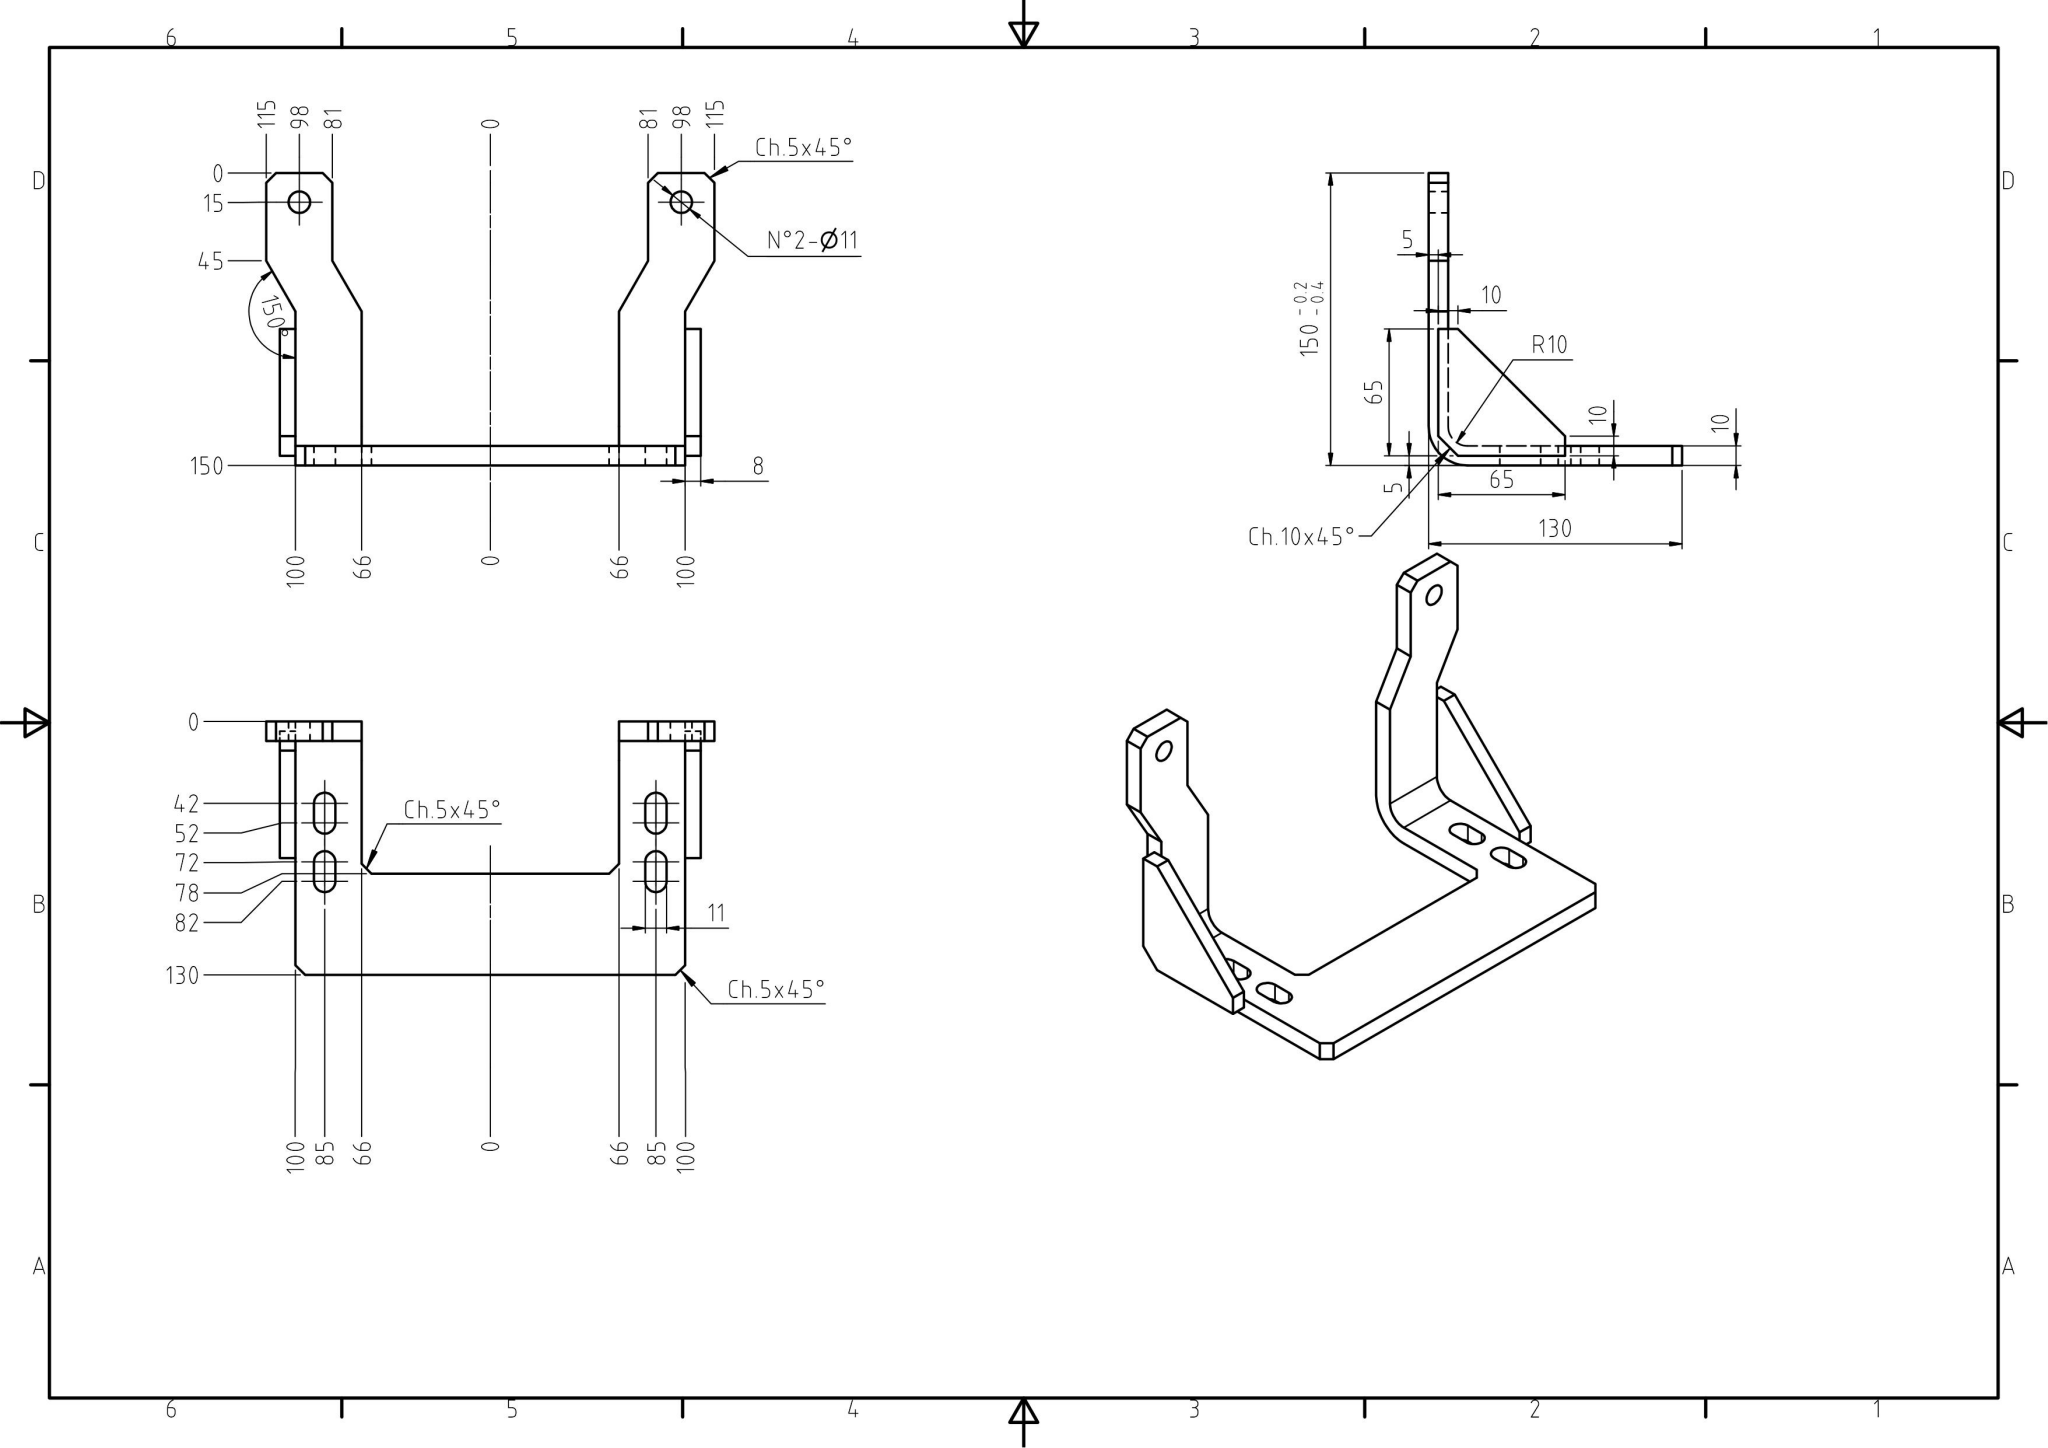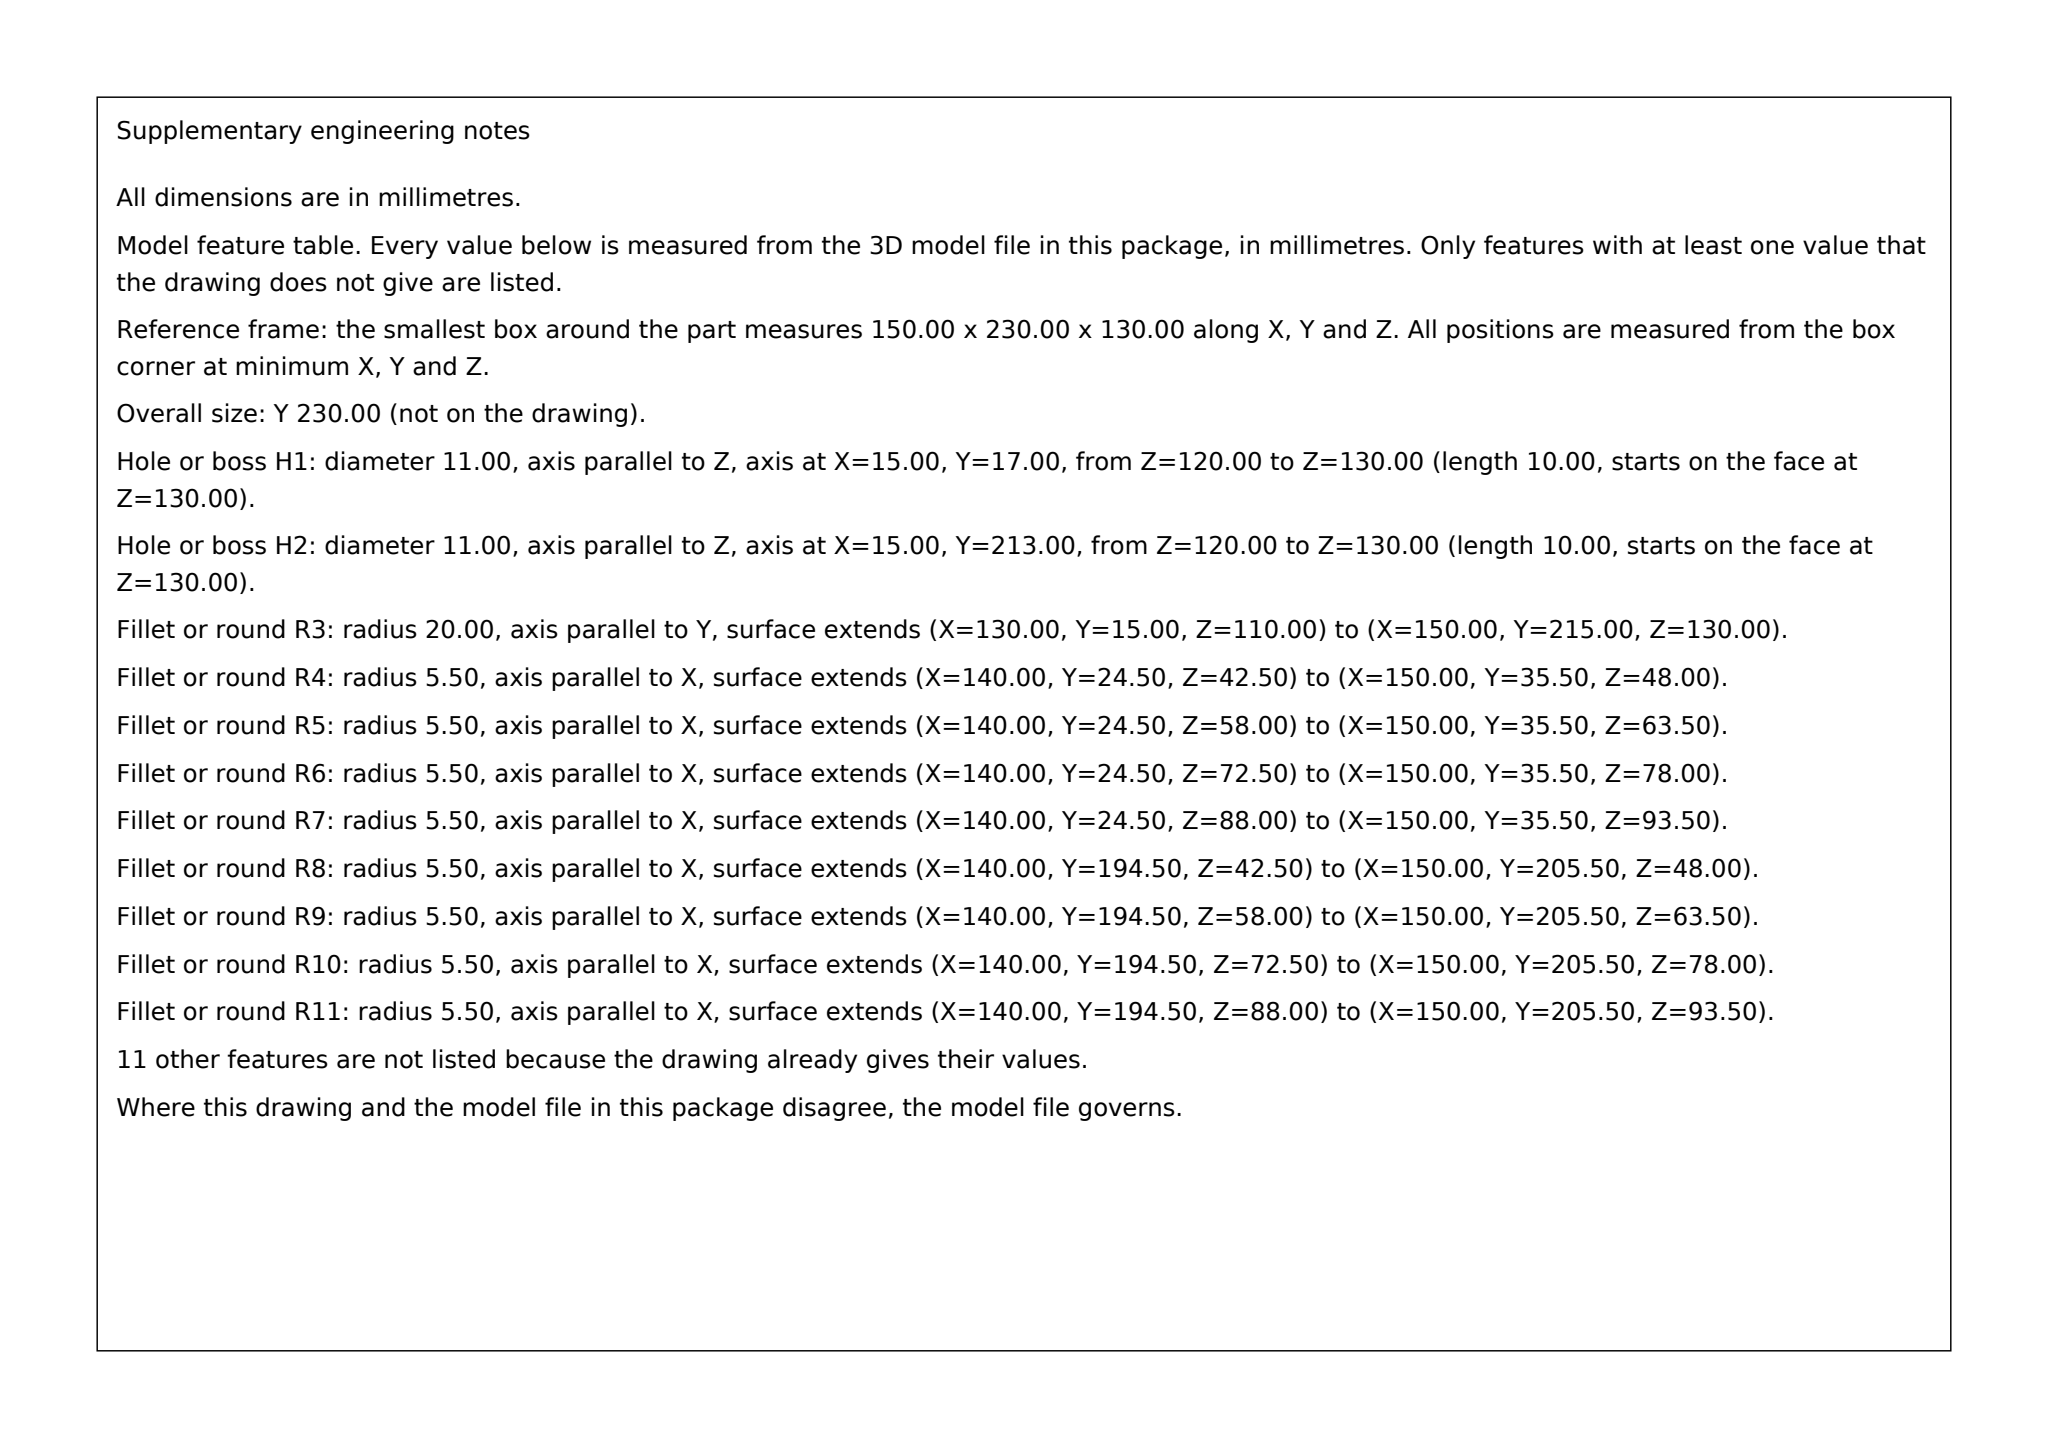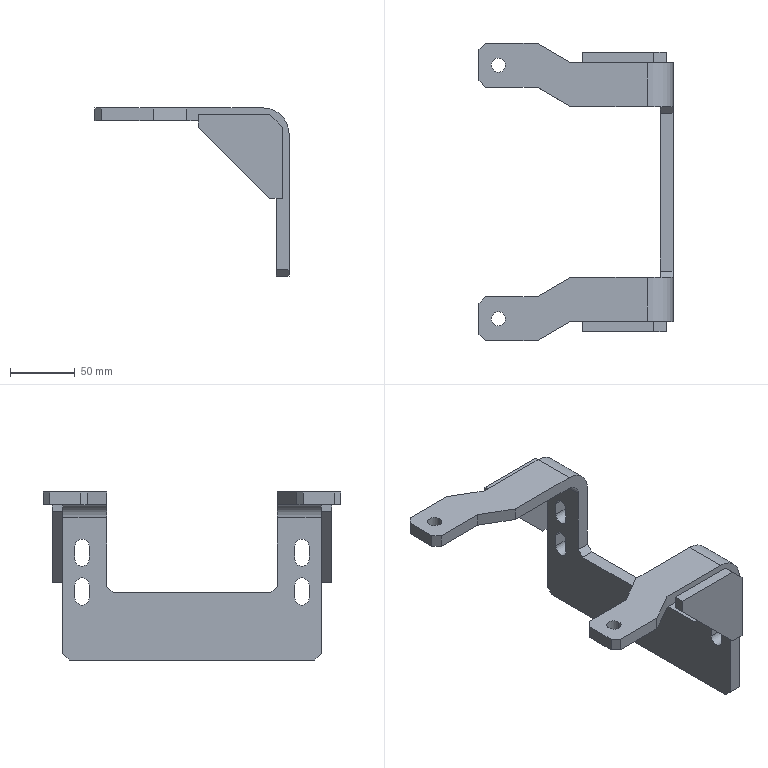Part | SolidWorks | mm | 1 solid | 70 faces | box 150 x 230 x 130 mm | volume 279860 mm3 | plane 54 | cylinder 16 | commonest cylinder face diameters 11 x12 40 x2 20 x2